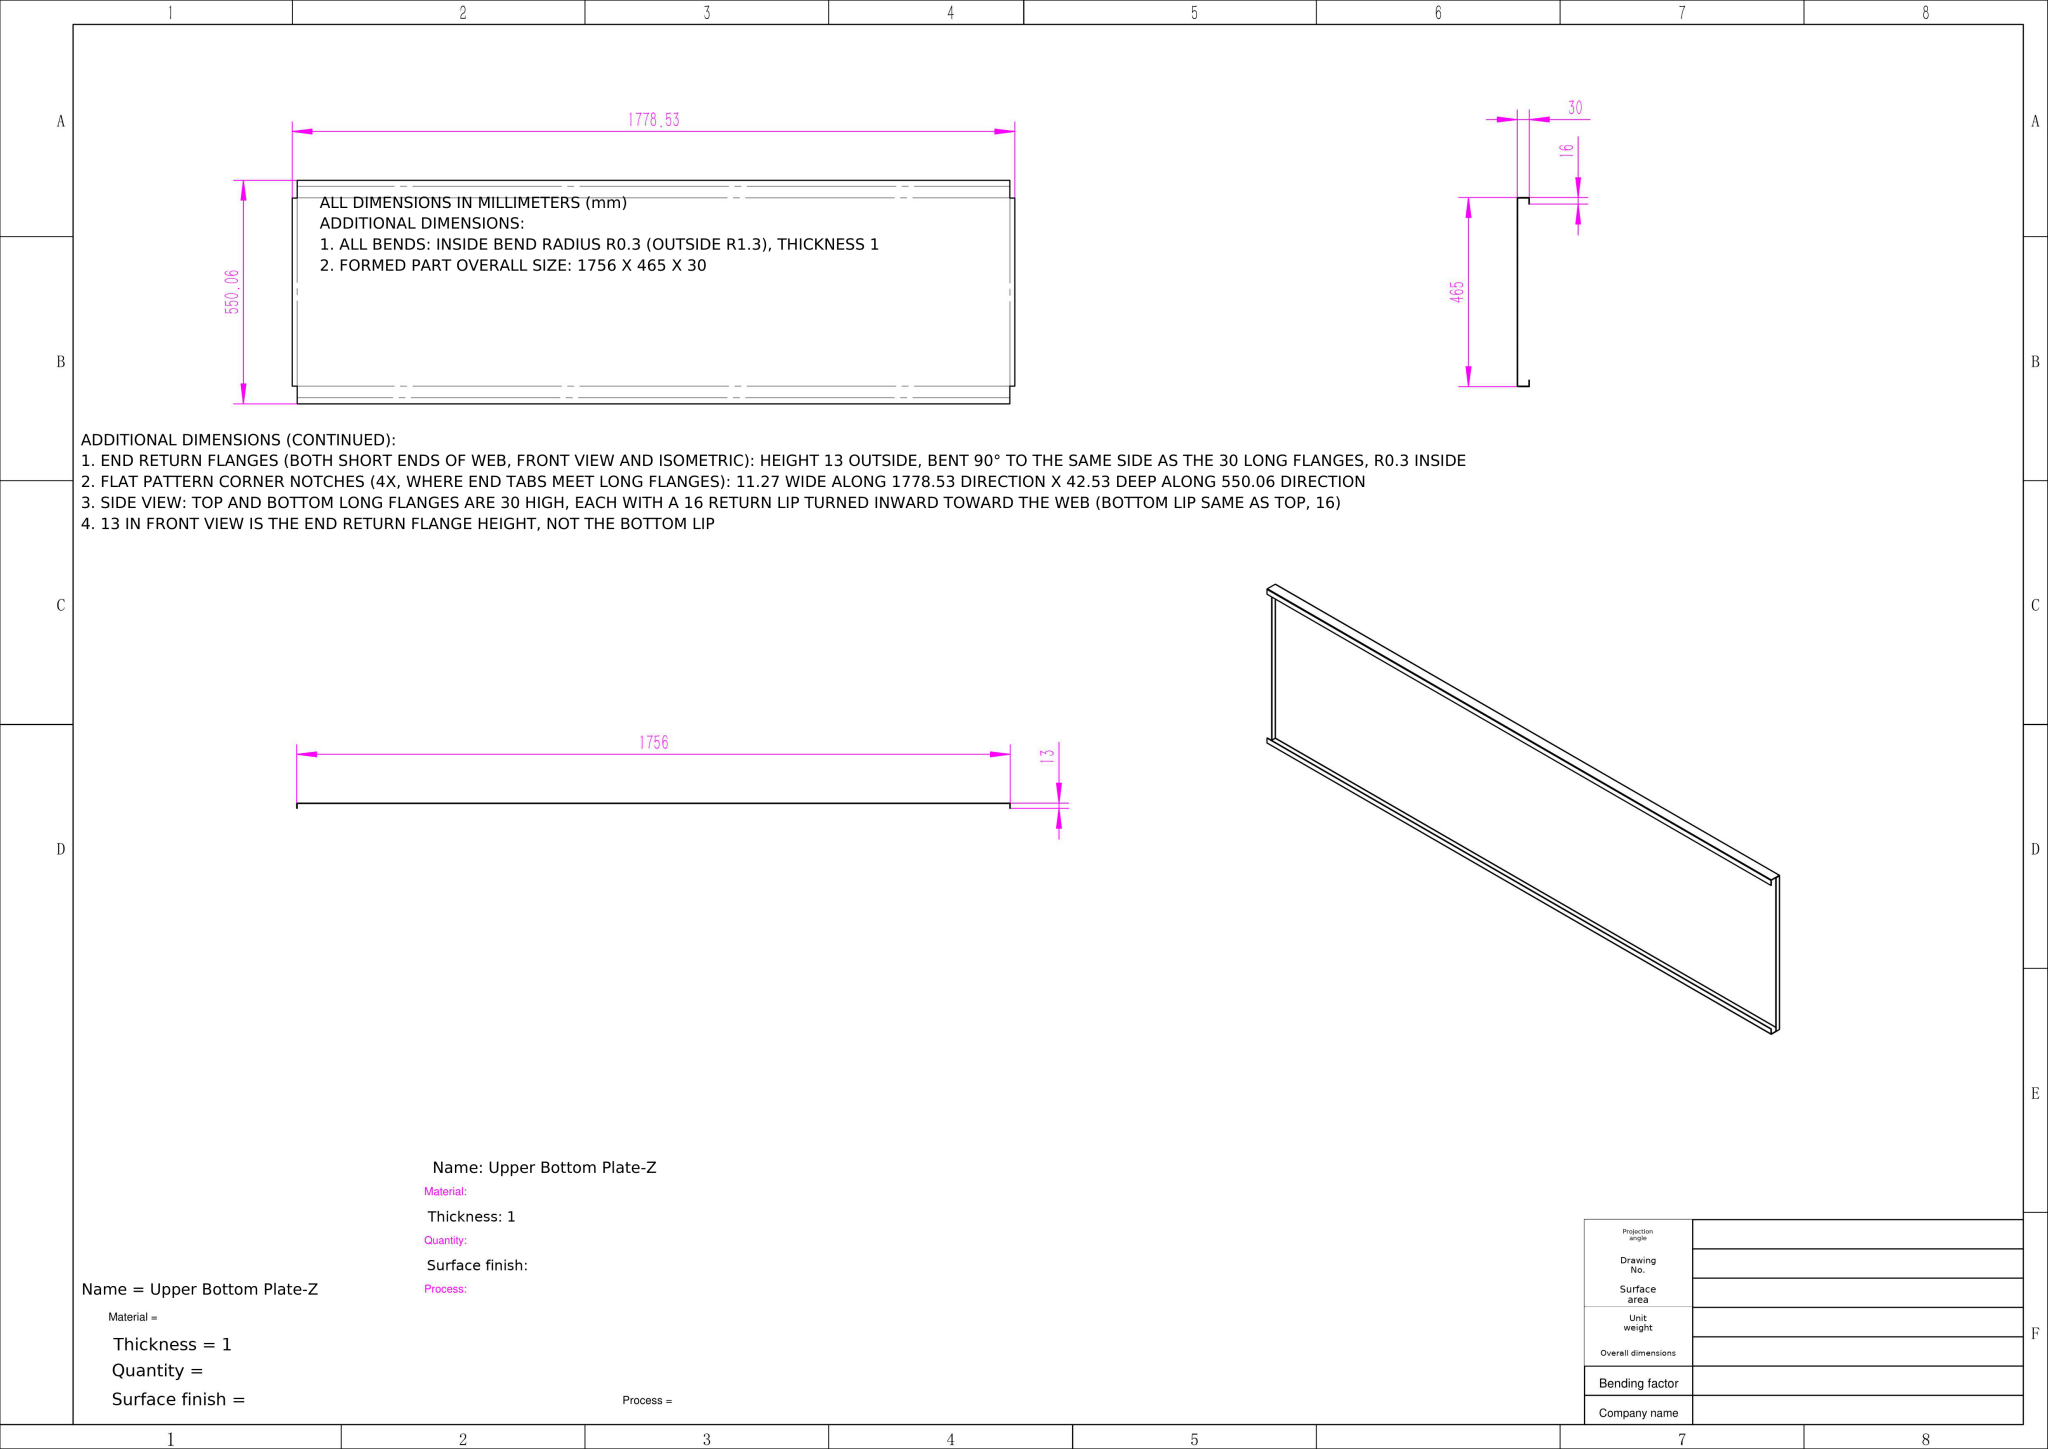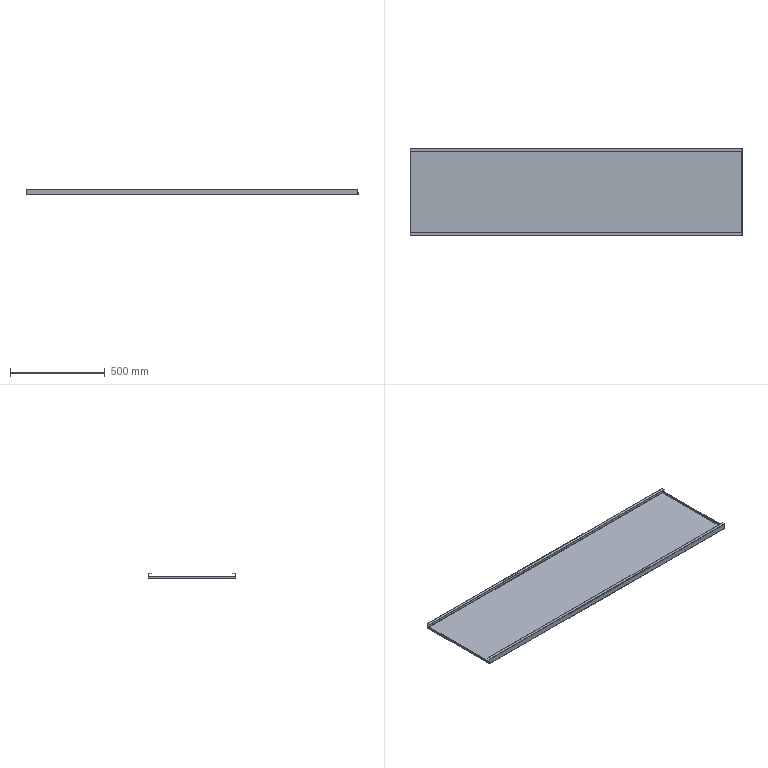Part | NX | mm | 1 solid | 58 faces | box 1756 x 465 x 30 mm | volume 979258 mm3 | plane 46 | cylinder 12 | commonest cylinder face diameters 2.6 x6 0.6 x6